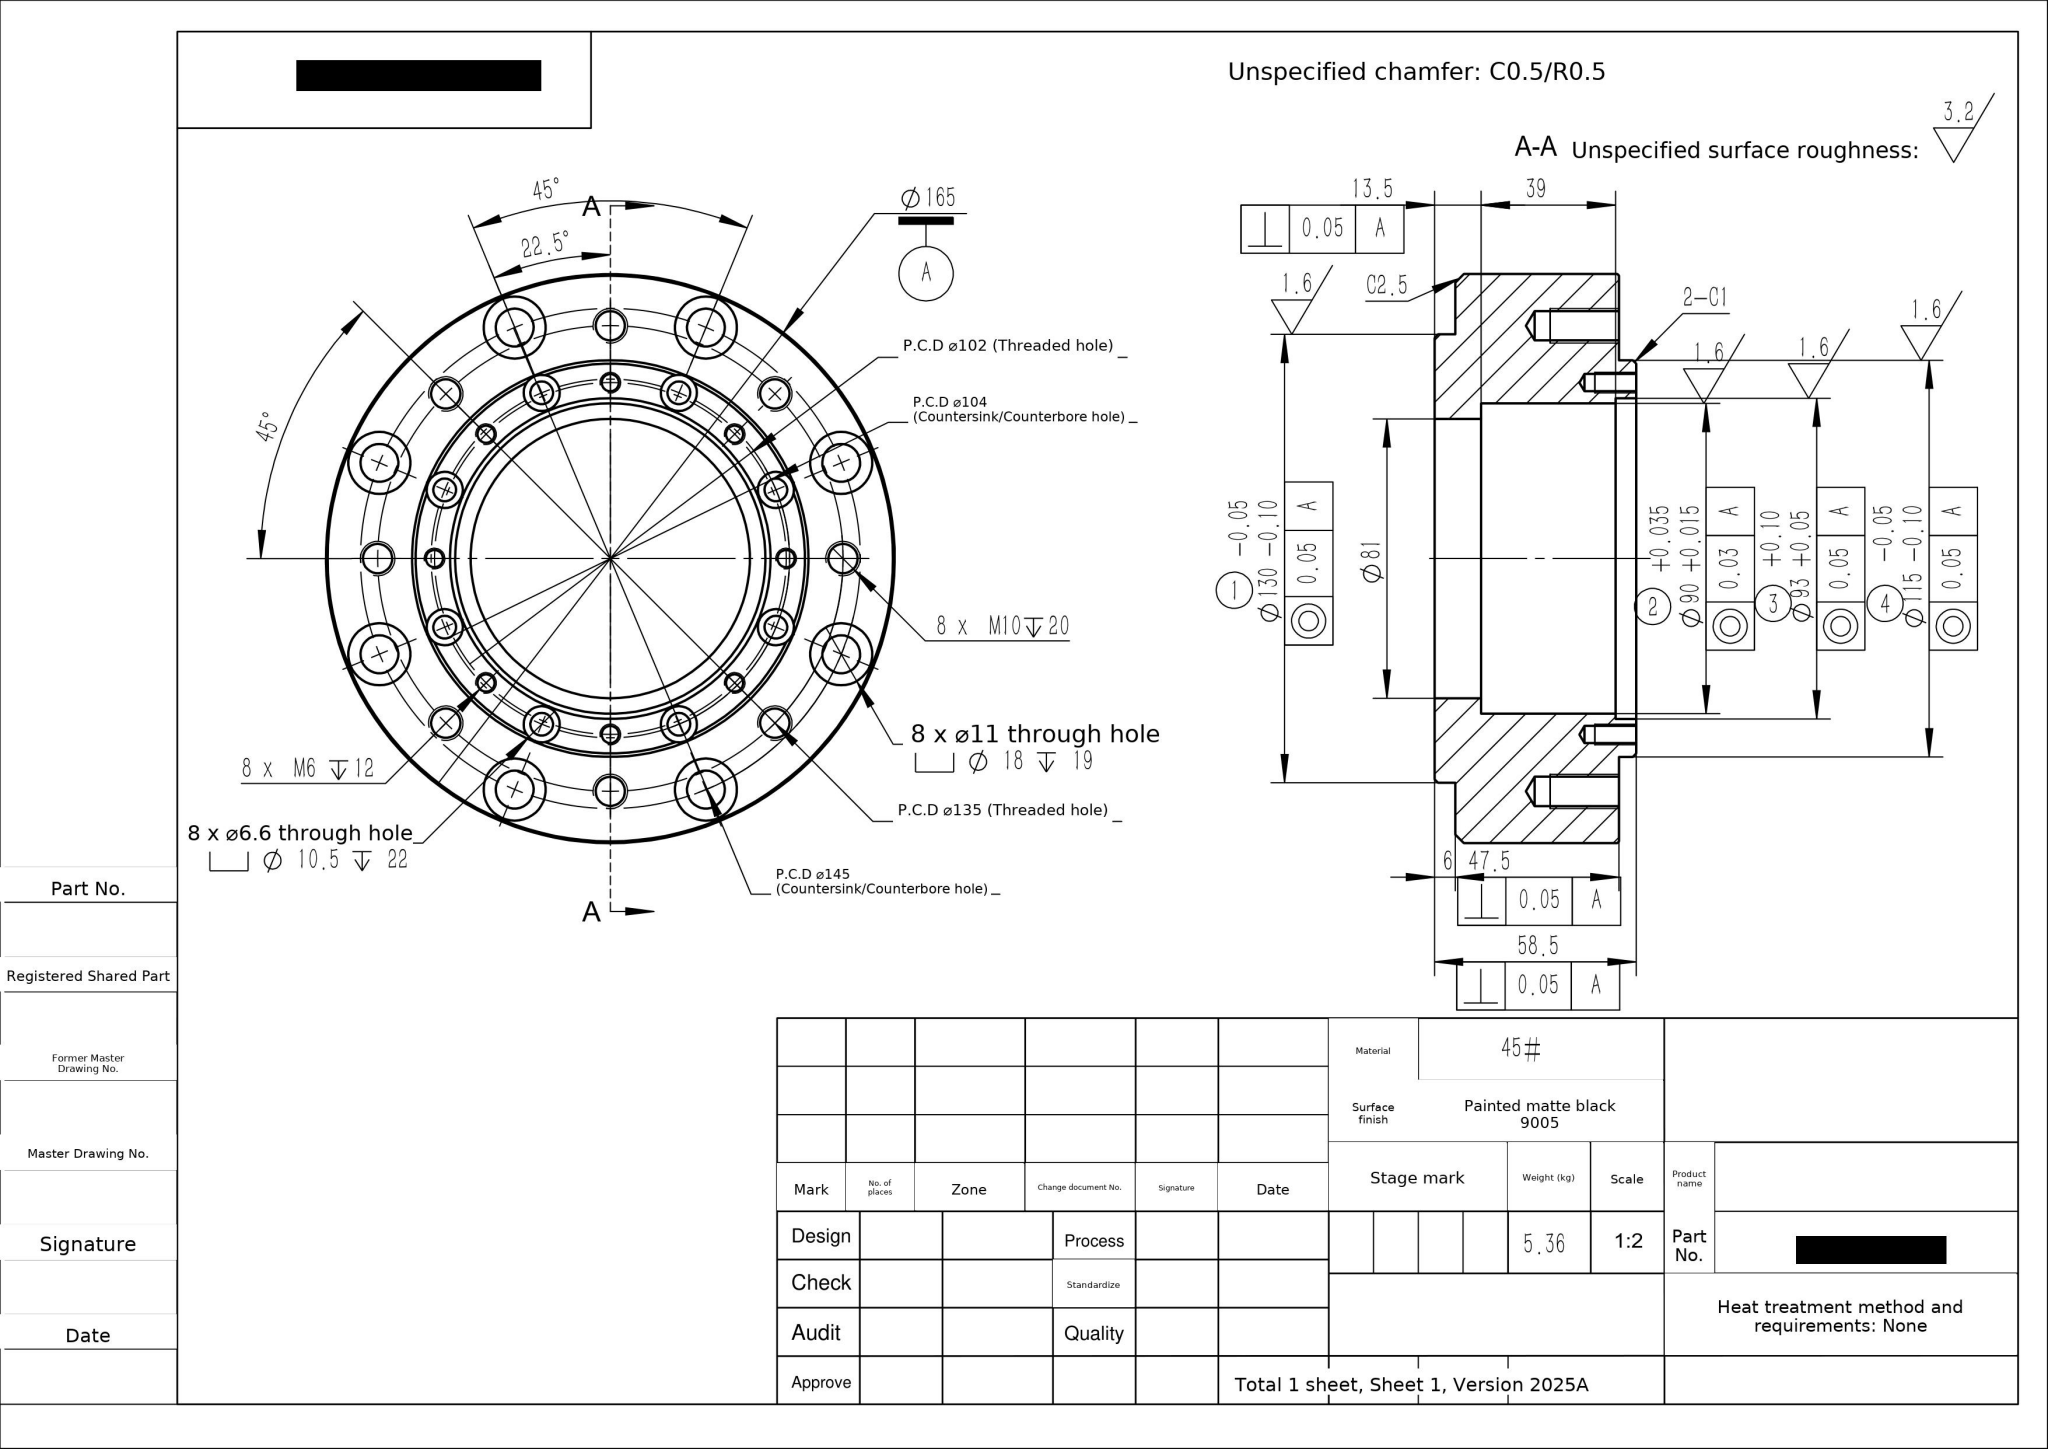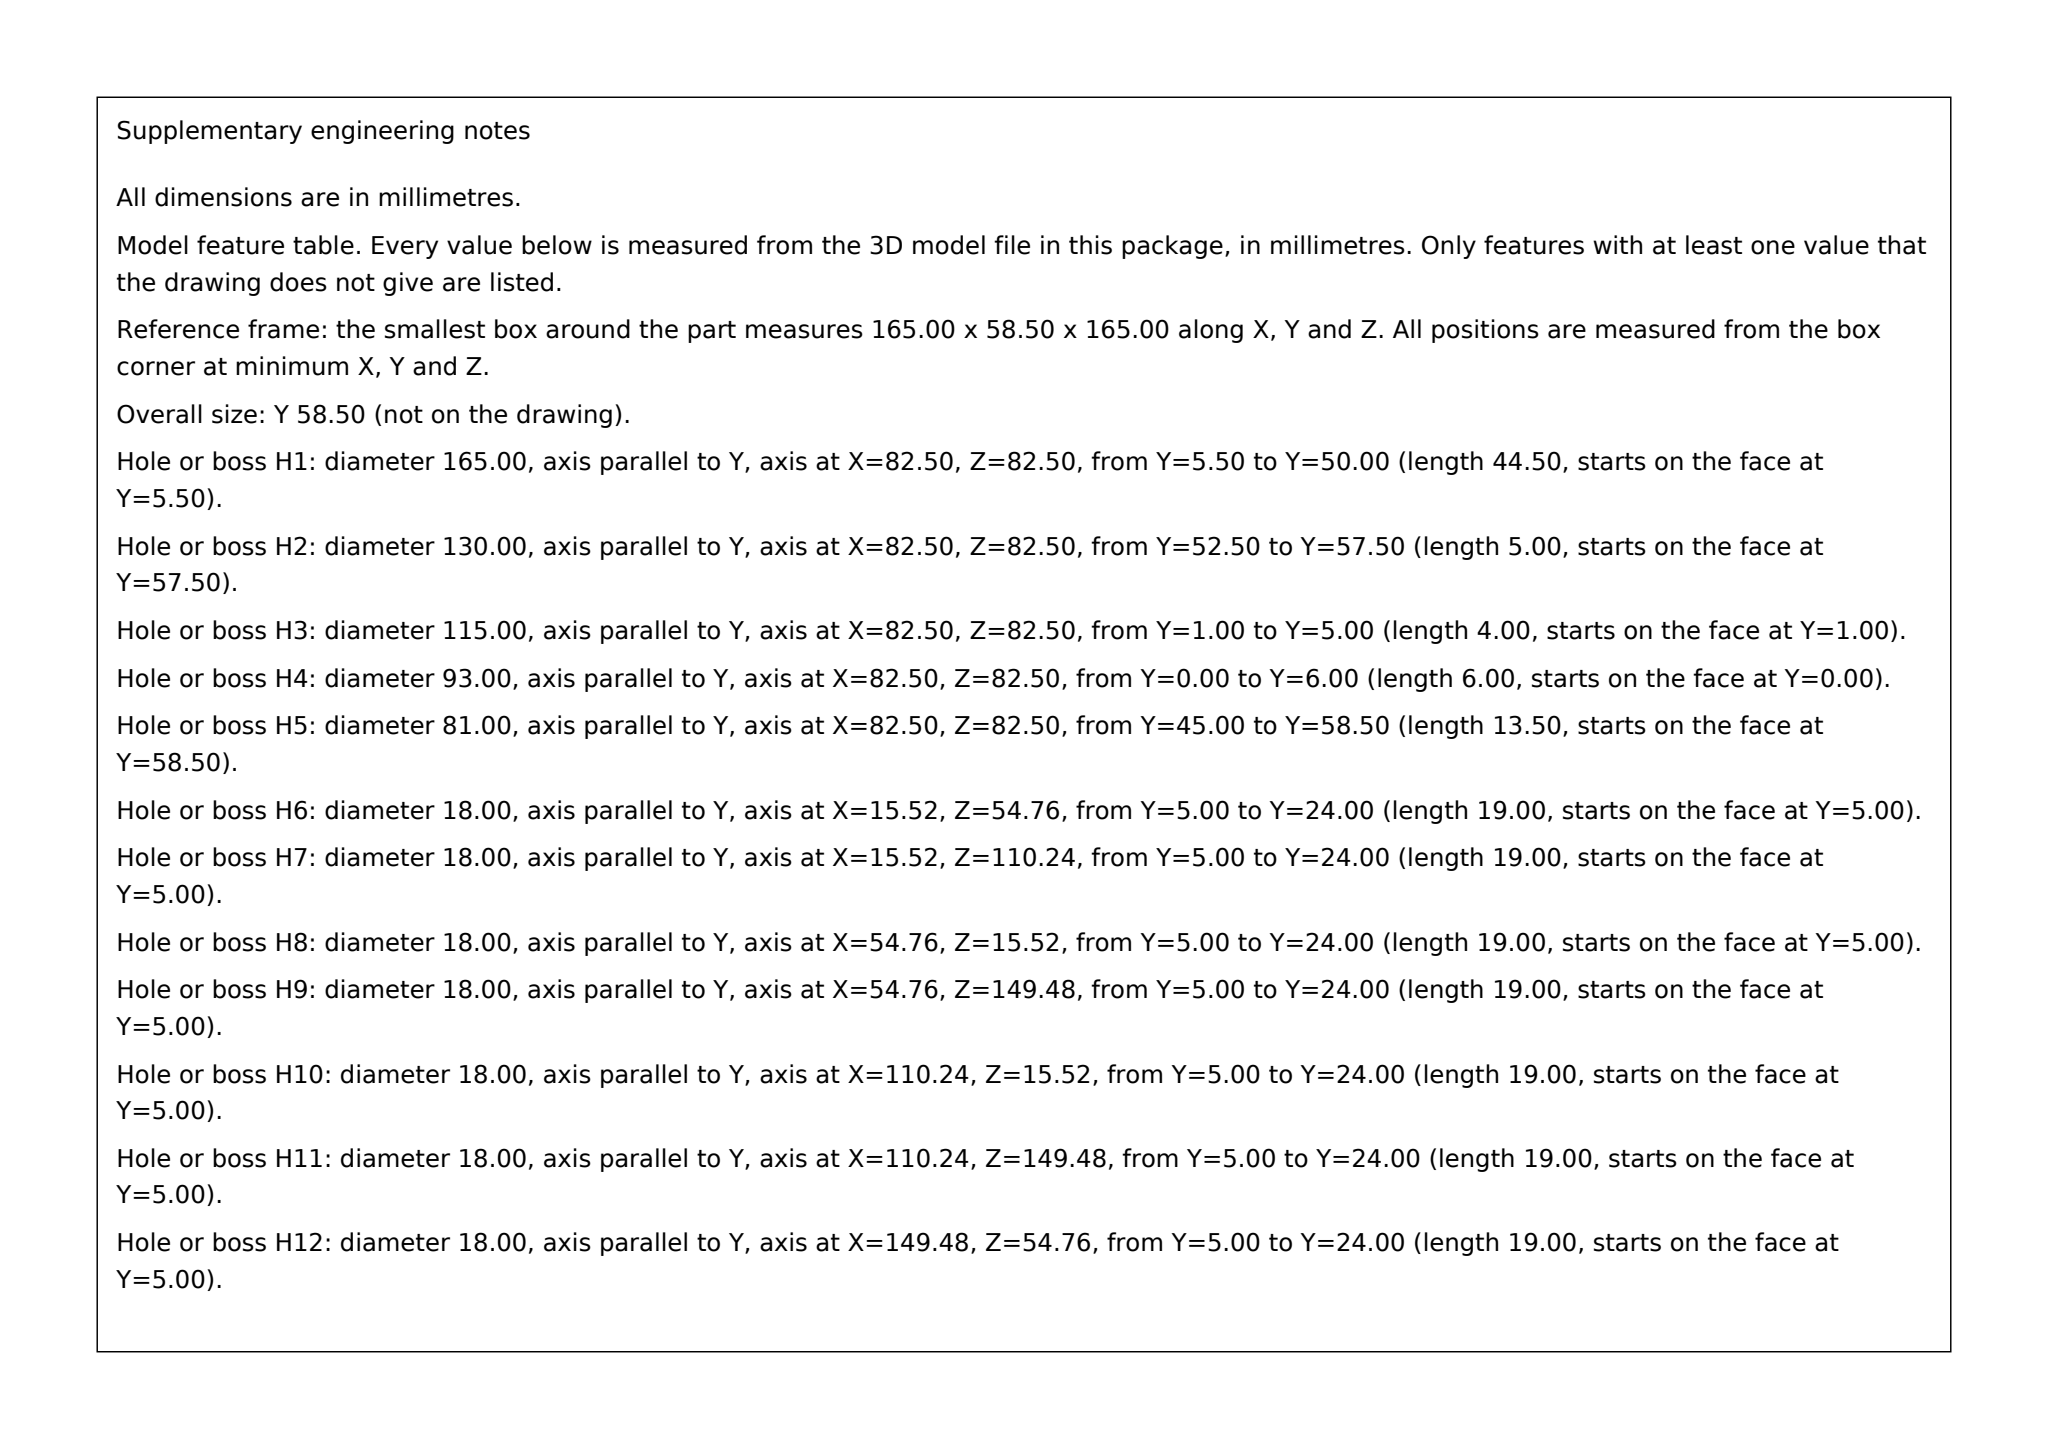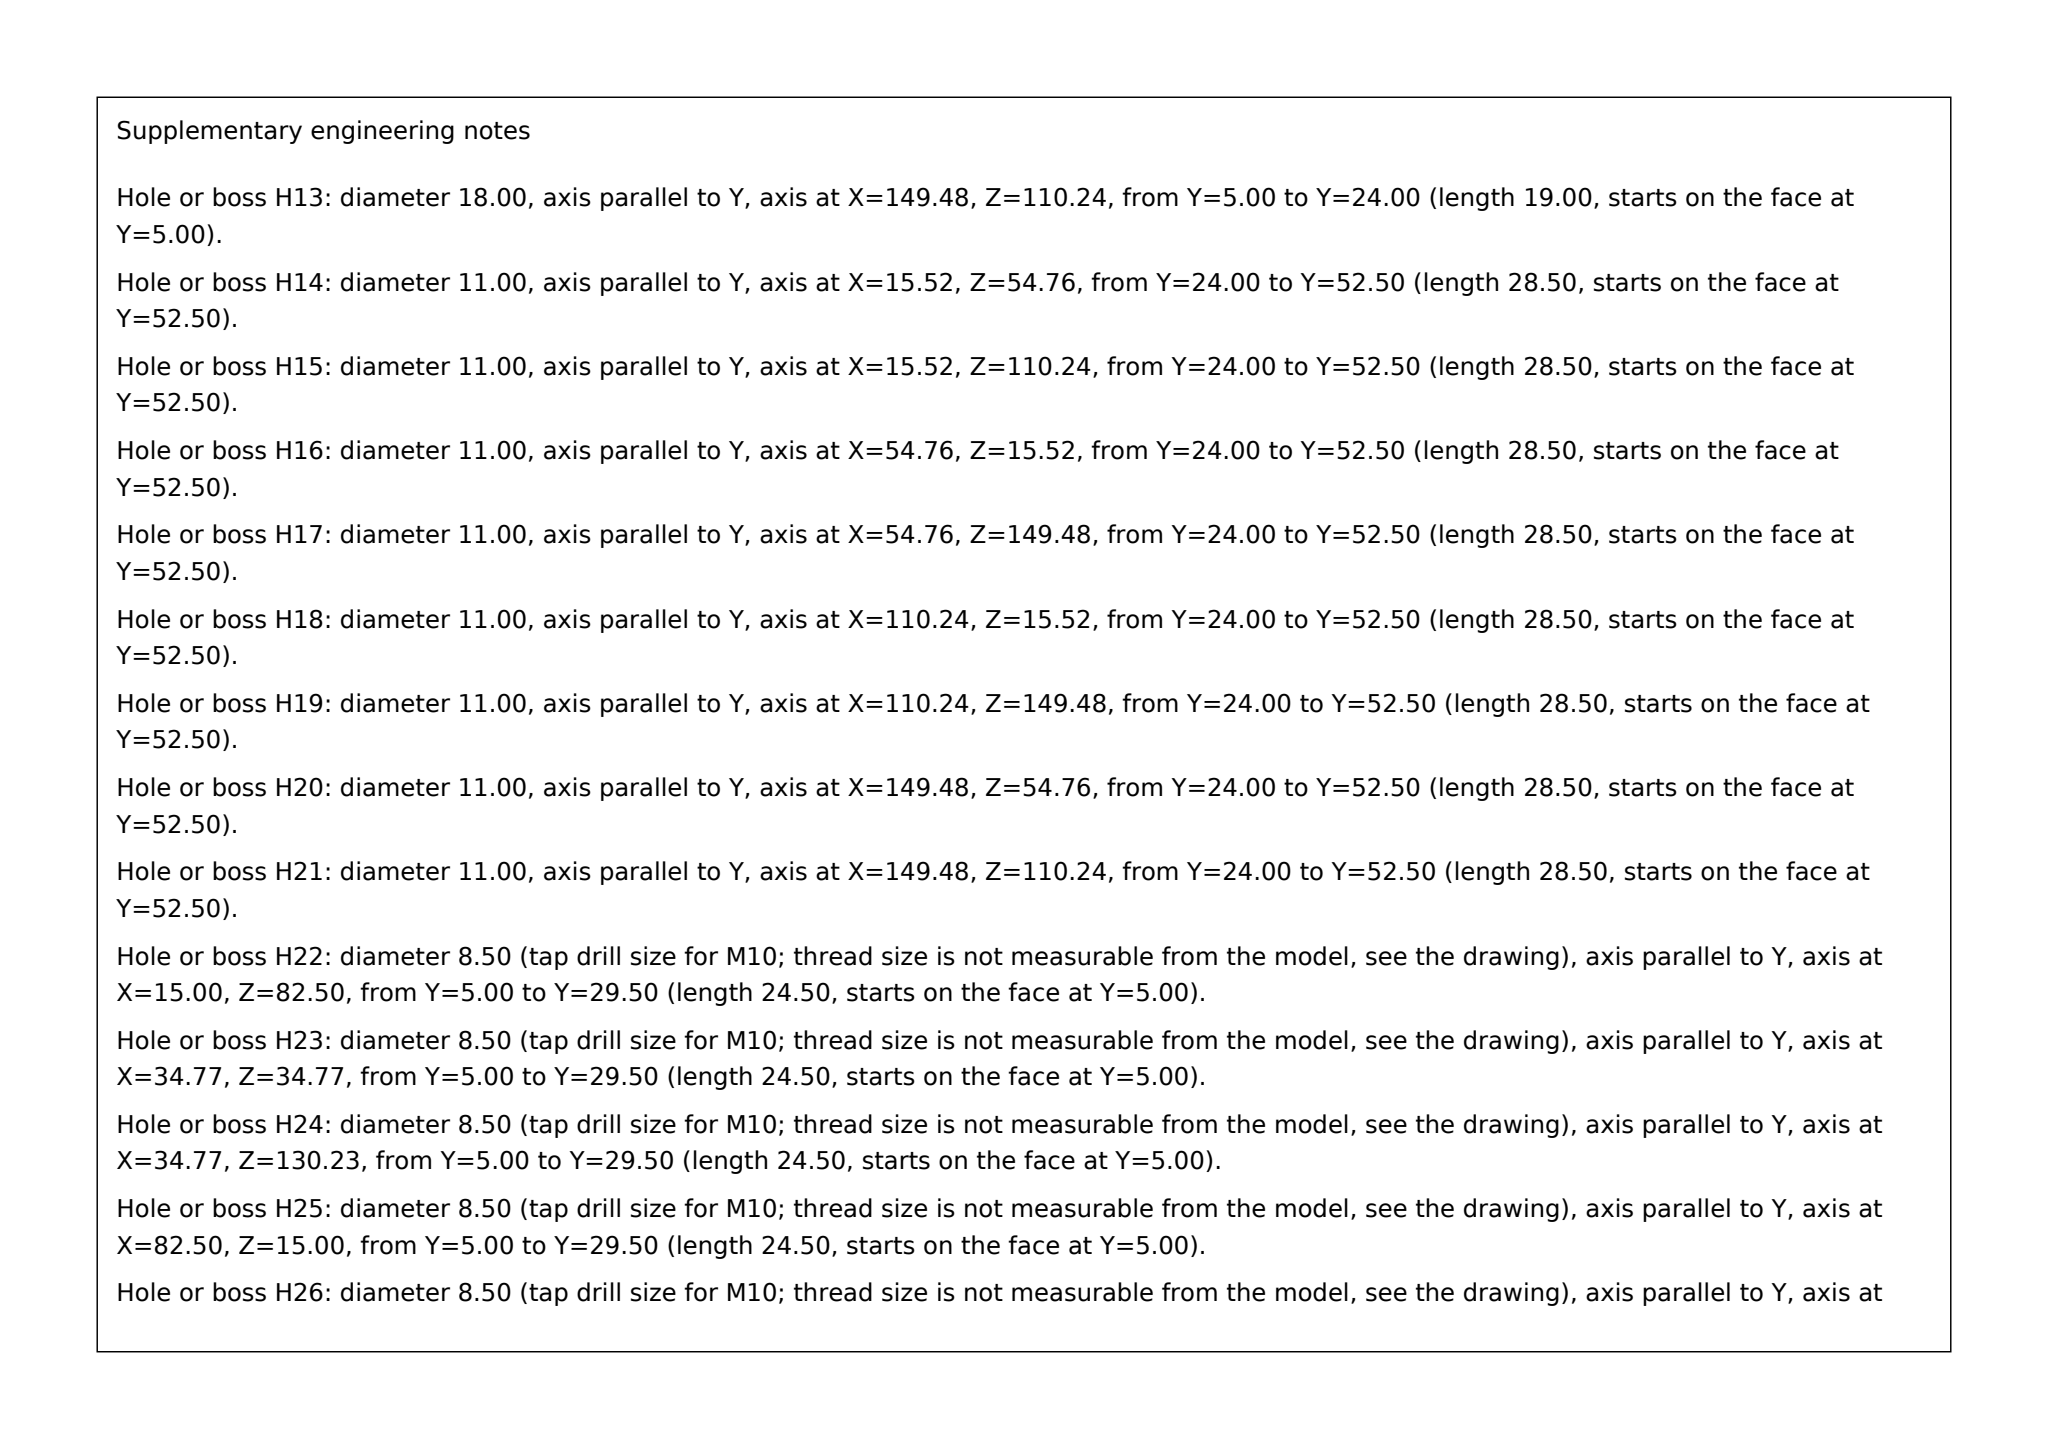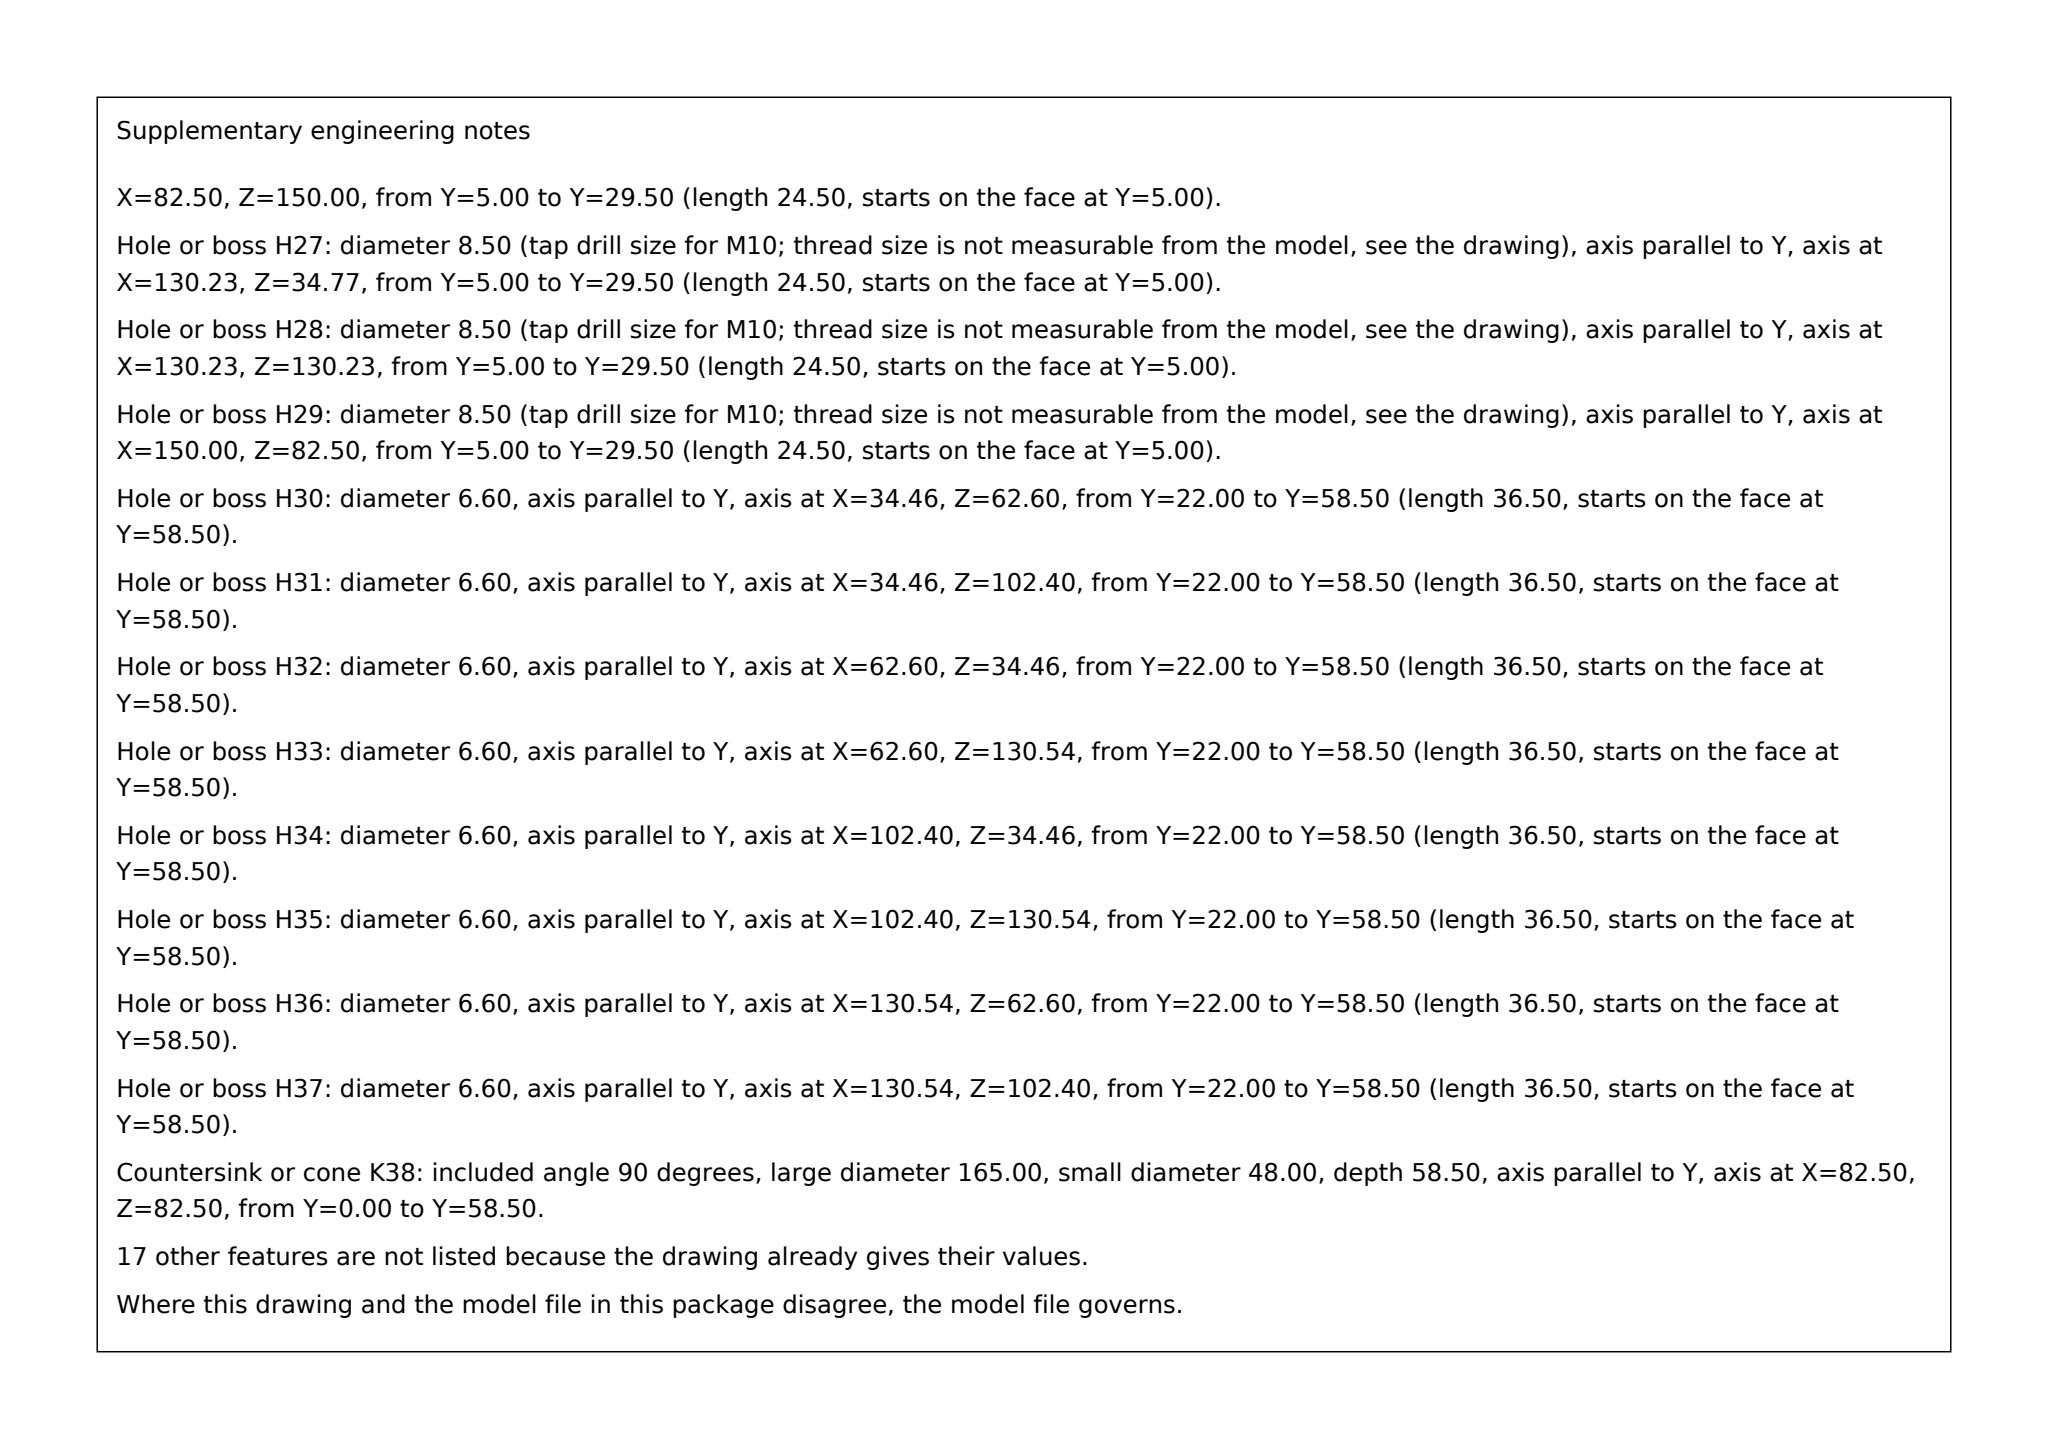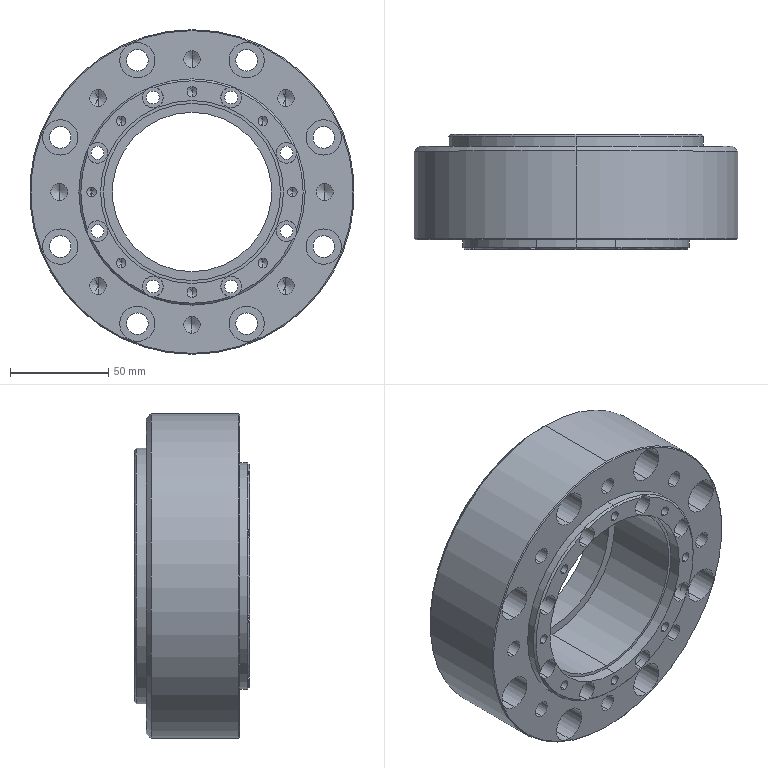Part | SolidWorks | mm | material 45# | 1 solid | 170 faces | box 165 x 58.5 x 165 mm | volume 687247 mm3 | cylinder 108 | cone 40 | plane 22 | commonest cylinder face diameters 5 x16 8.5 x16 10.5 x16 6.6 x16 18 x16 11 x16 81 x2 93 x2